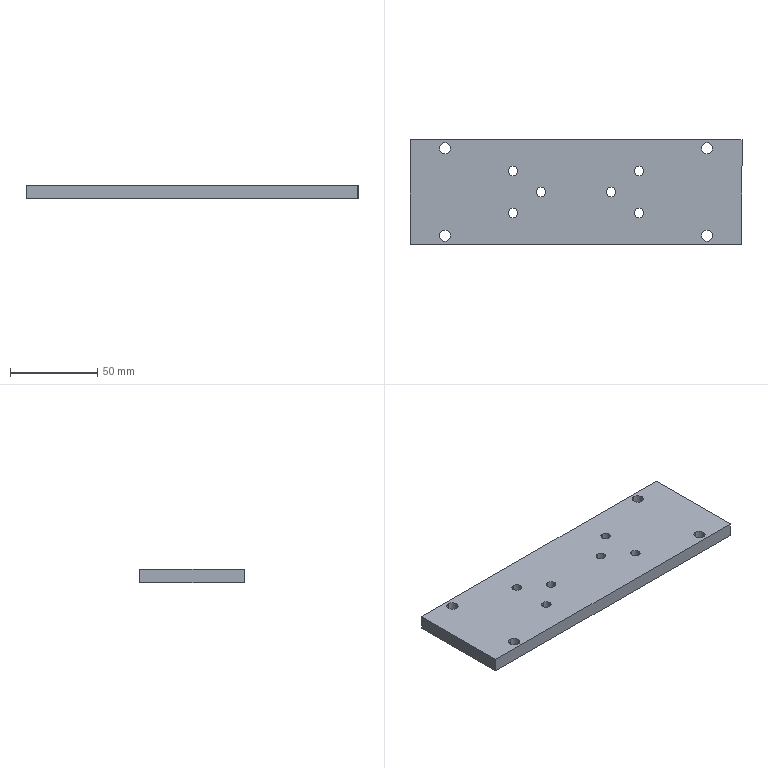Component | SolidWorks | JQ-2-0-001-1 | 1 solid | 26 faces | box 190 x 60 x 8 mm | volume 89071 mm3 | cylinder 20 | plane 6 | commonest cylinder face diameters 5.4 x12 6.4 x8
build123d program:
from build123d import *

# Parameters (mm, degrees)
SKETCH1_W           = 190
SKETCH1_H           = 8
BOSS_EXTRUDE1_DEPTH = 60
SKETCH7_R           = 3.2
CUT_EXTRUDE2_DEPTH  = 200.409
SKETCH8_R           = 2.7
CUT_EXTRUDE3_DEPTH  = 200.409


with BuildPart() as part:
    # Sketch1 → Boss-Extrude1 (new body)
    with BuildSketch(Plane.XY):
        with Locations((95, 4)):
            Rectangle(SKETCH1_W, SKETCH1_H)
    extrude(amount=BOSS_EXTRUDE1_DEPTH)

    # Sketch7 → Cut-Extrude2 (cut, through all)
    with BuildSketch(Plane(origin=(0, 8, 0), x_dir=(1, 0, 0), z_dir=(0, 1, 0))):
        with Locations(Location((170, -5, 0), (0, 0, 270))):
            Circle(SKETCH7_R)
        with Locations(Location((170, -55, 0), (0, 0, 270))):
            Circle(SKETCH7_R)
        with Locations(Location((20, -5, 0), (0, 0, 270))):
            Circle(SKETCH7_R)
        with Locations(Location((20, -55, 0), (0, 0, 270))):
            Circle(SKETCH7_R)
    extrude(amount=-CUT_EXTRUDE2_DEPTH, mode=Mode.SUBTRACT)

    # Sketch8 → Cut-Extrude3 (cut, through all)
    with BuildSketch(Plane.XZ):
        with Locations(Location((59, 42, 0), (0, 0, 270))):
            Circle(SKETCH8_R)
        with Locations(Location((131, 42, 0), (0, 0, 270))):
            Circle(SKETCH8_R)
        with Locations(Location((59, 18, 0), (0, 0, 270))):
            Circle(SKETCH8_R)
        with Locations(Location((131, 18, 0), (0, 0, 270))):
            Circle(SKETCH8_R)
        with Locations(Location((75, 30, 0), (0, 0, 270))):
            Circle(SKETCH8_R)
        with Locations(Location((115, 30, 0), (0, 0, 270))):
            Circle(SKETCH8_R)
    extrude(amount=-CUT_EXTRUDE3_DEPTH, mode=Mode.SUBTRACT)


solid = part.part

# Placed as in the assembly
solid = solid.moved(Location((-357.058, 59.339, -23.869), (90, 0, 0)))
STEP:
#1=CARTESIAN_POINT('',(-9.53,1.261,-0.9397));
#2=VERTEX_POINT('',#1);
#3=CARTESIAN_POINT('',(-9.53,1.049,-0.9397));
#4=VERTEX_POINT('',#3);
#5=CARTESIAN_POINT('',(-9.53,1.155,-0.9397));
#6=DIRECTION('',(0.,0.,1.));
#7=DIRECTION('',(0.,-1.,0.));
#8=AXIS2_PLACEMENT_3D('',#5,#6,#7);
#9=CIRCLE('',#8,0.1063);
#10=EDGE_CURVE('',#2,#4,#9,.T.);
#11=ORIENTED_EDGE('',*,*,#10,.F.);
#12=CARTESIAN_POINT('',(-9.53,1.261,-0.6248));
#13=VERTEX_POINT('',#12);
#14=CARTESIAN_POINT('',(-9.53,1.261,-0.9397));
#15=DIRECTION('',(0.,0.,1.));
#16=VECTOR('',#15,39.37);
#17=LINE('',#14,#16);
#18=EDGE_CURVE('',#2,#13,#17,.T.);
#19=ORIENTED_EDGE('',*,*,#18,.T.);
#20=CARTESIAN_POINT('',(-9.53,1.049,-0.6248));
#21=VERTEX_POINT('',#20);
#22=CARTESIAN_POINT('',(-9.53,1.155,-0.6248));
#23=DIRECTION('',(0.,0.,1.));
#24=DIRECTION('',(0.,-1.,0.));
#25=AXIS2_PLACEMENT_3D('',#22,#23,#24);
#26=CIRCLE('',#25,0.1063);
#27=EDGE_CURVE('',#13,#21,#26,.T.);
#28=ORIENTED_EDGE('',*,*,#27,.T.);
#29=CARTESIAN_POINT('',(-9.53,1.049,-0.9397));
#30=DIRECTION('',(0.,0.,1.));
#31=VECTOR('',#30,39.37);
#32=LINE('',#29,#31);
#33=EDGE_CURVE('',#4,#21,#32,.T.);
#34=ORIENTED_EDGE('',*,*,#33,.F.);
#35=EDGE_LOOP('',(#11,#19,#28,#34));
#36=FACE_OUTER_BOUND('',#35,.T.);
#37=CARTESIAN_POINT('',(-9.53,1.155,-0.9397));
#38=DIRECTION('',(0.,0.,1.));
#39=DIRECTION('',(0.,-1.,0.));
#40=AXIS2_PLACEMENT_3D('',#37,#38,#39);
#41=CYLINDRICAL_SURFACE('',#40,0.1063);
#42=ADVANCED_FACE('',(#36),#41,.F.);
#43=CARTESIAN_POINT('',(-11.105,1.261,-0.9397));
#44=VERTEX_POINT('',#43);
#45=CARTESIAN_POINT('',(-11.105,1.049,-0.9397));
#46=VERTEX_POINT('',#45);
#47=CARTESIAN_POINT('',(-11.105,1.155,-0.9397));
#48=DIRECTION('',(0.,0.,1.));
#49=DIRECTION('',(0.,-1.,0.));
#50=AXIS2_PLACEMENT_3D('',#47,#48,#49);
#51=CIRCLE('',#50,0.1063);
#52=EDGE_CURVE('',#44,#46,#51,.T.);
#53=ORIENTED_EDGE('',*,*,#52,.F.);
#54=CARTESIAN_POINT('',(-11.105,1.261,-0.6248));
#55=VERTEX_POINT('',#54);
#56=CARTESIAN_POINT('',(-11.105,1.261,-0.9397));
#57=DIRECTION('',(0.,0.,1.));
#58=VECTOR('',#57,39.37);
#59=LINE('',#56,#58);
#60=EDGE_CURVE('',#44,#55,#59,.T.);
#61=ORIENTED_EDGE('',*,*,#60,.T.);
#62=CARTESIAN_POINT('',(-11.105,1.049,-0.6248));
#63=VERTEX_POINT('',#62);
#64=CARTESIAN_POINT('',(-11.105,1.155,-0.6248));
#65=DIRECTION('',(0.,0.,1.));
#66=DIRECTION('',(0.,-1.,0.));
#67=AXIS2_PLACEMENT_3D('',#64,#65,#66);
#68=CIRCLE('',#67,0.1063);
#69=EDGE_CURVE('',#55,#63,#68,.T.);
#70=ORIENTED_EDGE('',*,*,#69,.T.);
#71=CARTESIAN_POINT('',(-11.105,1.049,-0.9397));
#72=DIRECTION('',(0.,0.,1.));
#73=VECTOR('',#72,39.37);
#74=LINE('',#71,#73);
#75=EDGE_CURVE('',#46,#63,#74,.T.);
#76=ORIENTED_EDGE('',*,*,#75,.F.);
#77=EDGE_LOOP('',(#53,#61,#70,#76));
#78=FACE_OUTER_BOUND('',#77,.T.);
#79=CARTESIAN_POINT('',(-11.105,1.155,-0.9397));
#80=DIRECTION('',(0.,0.,1.));
#81=DIRECTION('',(0.,-1.,0.));
#82=AXIS2_PLACEMENT_3D('',#79,#80,#81);
#83=CYLINDRICAL_SURFACE('',#82,0.1063);
#84=ADVANCED_FACE('',(#78),#83,.F.);
#85=CARTESIAN_POINT('',(-8.9,0.7889,-0.9397));
#86=VERTEX_POINT('',#85);
#87=CARTESIAN_POINT('',(-8.9,0.5763,-0.9397));
#88=VERTEX_POINT('',#87);
#89=CARTESIAN_POINT('',(-8.9,0.6826,-0.9397));
#90=DIRECTION('',(0.,0.,1.));
#91=DIRECTION('',(0.,-1.,0.));
#92=AXIS2_PLACEMENT_3D('',#89,#90,#91);
#93=CIRCLE('',#92,0.1063);
#94=EDGE_CURVE('',#86,#88,#93,.T.);
#95=ORIENTED_EDGE('',*,*,#94,.F.);
#96=CARTESIAN_POINT('',(-8.9,0.7889,-0.6248));
#97=VERTEX_POINT('',#96);
#98=CARTESIAN_POINT('',(-8.9,0.7889,-0.9397));
#99=DIRECTION('',(0.,0.,1.));
#100=VECTOR('',#99,39.37);
#101=LINE('',#98,#100);
#102=EDGE_CURVE('',#86,#97,#101,.T.);
#103=ORIENTED_EDGE('',*,*,#102,.T.);
#104=CARTESIAN_POINT('',(-8.9,0.5763,-0.6248));
#105=VERTEX_POINT('',#104);
#106=CARTESIAN_POINT('',(-8.9,0.6826,-0.6248));
#107=DIRECTION('',(0.,0.,1.));
#108=DIRECTION('',(0.,-1.,0.));
#109=AXIS2_PLACEMENT_3D('',#106,#107,#108);
#110=CIRCLE('',#109,0.1063);
#111=EDGE_CURVE('',#97,#105,#110,.T.);
#112=ORIENTED_EDGE('',*,*,#111,.T.);
#113=CARTESIAN_POINT('',(-8.9,0.5763,-0.9397));
#114=DIRECTION('',(0.,0.,1.));
#115=VECTOR('',#114,39.37);
#116=LINE('',#113,#115);
#117=EDGE_CURVE('',#88,#105,#116,.T.);
#118=ORIENTED_EDGE('',*,*,#117,.F.);
#119=EDGE_LOOP('',(#95,#103,#112,#118));
#120=FACE_OUTER_BOUND('',#119,.T.);
#121=CARTESIAN_POINT('',(-8.9,0.6826,-0.9397));
#122=DIRECTION('',(0.,0.,1.));
#123=DIRECTION('',(0.,-1.,0.));
#124=AXIS2_PLACEMENT_3D('',#121,#122,#123);
#125=CYLINDRICAL_SURFACE('',#124,0.1063);
#126=ADVANCED_FACE('',(#120),#125,.F.);
#127=CARTESIAN_POINT('',(-11.735,0.7889,-0.9397));
#128=VERTEX_POINT('',#127);
#129=CARTESIAN_POINT('',(-11.735,0.5763,-0.9397));
#130=VERTEX_POINT('',#129);
#131=CARTESIAN_POINT('',(-11.735,0.6826,-0.9397));
#132=DIRECTION('',(0.,0.,1.));
#133=DIRECTION('',(0.,-1.,0.));
#134=AXIS2_PLACEMENT_3D('',#131,#132,#133);
#135=CIRCLE('',#134,0.1063);
#136=EDGE_CURVE('',#128,#130,#135,.T.);
#137=ORIENTED_EDGE('',*,*,#136,.F.);
#138=CARTESIAN_POINT('',(-11.735,0.7889,-0.6248));
#139=VERTEX_POINT('',#138);
#140=CARTESIAN_POINT('',(-11.735,0.7889,-0.9397));
#141=DIRECTION('',(0.,0.,1.));
#142=VECTOR('',#141,39.37);
#143=LINE('',#140,#142);
#144=EDGE_CURVE('',#128,#139,#143,.T.);
#145=ORIENTED_EDGE('',*,*,#144,.T.);
#146=CARTESIAN_POINT('',(-11.735,0.5763,-0.6248));
#147=VERTEX_POINT('',#146);
#148=CARTESIAN_POINT('',(-11.735,0.6826,-0.6248));
#149=DIRECTION('',(0.,0.,1.));
#150=DIRECTION('',(0.,-1.,0.));
#151=AXIS2_PLACEMENT_3D('',#148,#149,#150);
#152=CIRCLE('',#151,0.1063);
#153=EDGE_CURVE('',#139,#147,#152,.T.);
#154=ORIENTED_EDGE('',*,*,#153,.T.);
#155=CARTESIAN_POINT('',(-11.735,0.5763,-0.9397));
#156=DIRECTION('',(0.,0.,1.));
#157=VECTOR('',#156,39.37);
#158=LINE('',#155,#157);
#159=EDGE_CURVE('',#130,#147,#158,.T.);
#160=ORIENTED_EDGE('',*,*,#159,.F.);
#161=EDGE_LOOP('',(#137,#145,#154,#160));
#162=FACE_OUTER_BOUND('',#161,.T.);
#163=CARTESIAN_POINT('',(-11.735,0.6826,-0.9397));
#164=DIRECTION('',(0.,0.,1.));
#165=DIRECTION('',(0.,-1.,0.));
#166=AXIS2_PLACEMENT_3D('',#163,#164,#165);
#167=CYLINDRICAL_SURFACE('',#166,0.1063);
#168=ADVANCED_FACE('',(#162),#167,.F.);
#169=CARTESIAN_POINT('',(-8.9,1.734,-0.9397));
#170=VERTEX_POINT('',#169);
#171=CARTESIAN_POINT('',(-8.9,1.521,-0.9397));
#172=VERTEX_POINT('',#171);
#173=CARTESIAN_POINT('',(-8.9,1.628,-0.9397));
#174=DIRECTION('',(0.,0.,1.));
#175=DIRECTION('',(0.,-1.,0.));
#176=AXIS2_PLACEMENT_3D('',#173,#174,#175);
#177=CIRCLE('',#176,0.1063);
#178=EDGE_CURVE('',#170,#172,#177,.T.);
#179=ORIENTED_EDGE('',*,*,#178,.F.);
#180=CARTESIAN_POINT('',(-8.9,1.734,-0.6248));
#181=VERTEX_POINT('',#180);
#182=CARTESIAN_POINT('',(-8.9,1.734,-0.9397));
#183=DIRECTION('',(0.,0.,1.));
#184=VECTOR('',#183,39.37);
#185=LINE('',#182,#184);
#186=EDGE_CURVE('',#170,#181,#185,.T.);
#187=ORIENTED_EDGE('',*,*,#186,.T.);
#188=CARTESIAN_POINT('',(-8.9,1.521,-0.6248));
#189=VERTEX_POINT('',#188);
#190=CARTESIAN_POINT('',(-8.9,1.628,-0.6248));
#191=DIRECTION('',(0.,0.,1.));
#192=DIRECTION('',(0.,-1.,0.));
#193=AXIS2_PLACEMENT_3D('',#190,#191,#192);
#194=CIRCLE('',#193,0.1063);
#195=EDGE_CURVE('',#181,#189,#194,.T.);
#196=ORIENTED_EDGE('',*,*,#195,.T.);
#197=CARTESIAN_POINT('',(-8.9,1.521,-0.9397));
#198=DIRECTION('',(0.,0.,1.));
#199=VECTOR('',#198,39.37);
#200=LINE('',#197,#199);
#201=EDGE_CURVE('',#172,#189,#200,.T.);
#202=ORIENTED_EDGE('',*,*,#201,.F.);
#203=EDGE_LOOP('',(#179,#187,#196,#202));
#204=FACE_OUTER_BOUND('',#203,.T.);
#205=CARTESIAN_POINT('',(-8.9,1.628,-0.9397));
#206=DIRECTION('',(0.,0.,1.));
#207=DIRECTION('',(0.,-1.,0.));
#208=AXIS2_PLACEMENT_3D('',#205,#206,#207);
#209=CYLINDRICAL_SURFACE('',#208,0.1063);
#210=ADVANCED_FACE('',(#204),#209,.F.);
#211=CARTESIAN_POINT('',(-11.735,1.734,-0.9397));
#212=VERTEX_POINT('',#211);
#213=CARTESIAN_POINT('',(-11.735,1.521,-0.9397));
#214=VERTEX_POINT('',#213);
#215=CARTESIAN_POINT('',(-11.735,1.628,-0.9397));
#216=DIRECTION('',(0.,0.,1.));
#217=DIRECTION('',(0.,-1.,0.));
#218=AXIS2_PLACEMENT_3D('',#215,#216,#217);
#219=CIRCLE('',#218,0.1063);
#220=EDGE_CURVE('',#212,#214,#219,.T.);
#221=ORIENTED_EDGE('',*,*,#220,.F.);
#222=CARTESIAN_POINT('',(-11.735,1.734,-0.6248));
#223=VERTEX_POINT('',#222);
#224=CARTESIAN_POINT('',(-11.735,1.734,-0.9397));
#225=DIRECTION('',(0.,0.,1.));
#226=VECTOR('',#225,39.37);
#227=LINE('',#224,#226);
#228=EDGE_CURVE('',#212,#223,#227,.T.);
#229=ORIENTED_EDGE('',*,*,#228,.T.);
#230=CARTESIAN_POINT('',(-11.735,1.521,-0.6248));
#231=VERTEX_POINT('',#230);
#232=CARTESIAN_POINT('',(-11.735,1.628,-0.6248));
#233=DIRECTION('',(0.,0.,1.));
#234=DIRECTION('',(0.,-1.,0.));
#235=AXIS2_PLACEMENT_3D('',#232,#233,#234);
#236=CIRCLE('',#235,0.1063);
#237=EDGE_CURVE('',#223,#231,#236,.T.);
#238=ORIENTED_EDGE('',*,*,#237,.T.);
#239=CARTESIAN_POINT('',(-11.735,1.521,-0.9397));
#240=DIRECTION('',(0.,0.,1.));
#241=VECTOR('',#240,39.37);
#242=LINE('',#239,#241);
#243=EDGE_CURVE('',#214,#231,#242,.T.);
#244=ORIENTED_EDGE('',*,*,#243,.F.);
#245=EDGE_LOOP('',(#221,#229,#238,#244));
#246=FACE_OUTER_BOUND('',#245,.T.);
#247=CARTESIAN_POINT('',(-11.735,1.628,-0.9397));
#248=DIRECTION('',(0.,0.,1.));
#249=DIRECTION('',(0.,-1.,0.));
#250=AXIS2_PLACEMENT_3D('',#247,#248,#249);
#251=CYLINDRICAL_SURFACE('',#250,0.1063);
#252=ADVANCED_FACE('',(#246),#251,.F.);
#253=CARTESIAN_POINT('',(-13.27,2.013,-0.6248));
#254=VERTEX_POINT('',#253);
#255=CARTESIAN_POINT('',(-13.27,2.265,-0.6248));
#256=VERTEX_POINT('',#255);
#257=CARTESIAN_POINT('',(-13.27,2.139,-0.6248));
#258=DIRECTION('',(-0.,-0.,-1.));
#259=DIRECTION('',(0.,1.,0.));
#260=AXIS2_PLACEMENT_3D('',#257,#258,#259);
#261=CIRCLE('',#260,0.126);
#262=EDGE_CURVE('',#254,#256,#261,.T.);
#263=ORIENTED_EDGE('',*,*,#262,.F.);
#264=CARTESIAN_POINT('',(-13.27,2.013,-0.9397));
#265=VERTEX_POINT('',#264);
#266=CARTESIAN_POINT('',(-13.27,2.013,-0.6248));
#267=DIRECTION('',(-0.,-0.,-1.));
#268=VECTOR('',#267,39.37);
#269=LINE('',#266,#268);
#270=EDGE_CURVE('',#254,#265,#269,.T.);
#271=ORIENTED_EDGE('',*,*,#270,.T.);
#272=CARTESIAN_POINT('',(-13.27,2.265,-0.9397));
#273=VERTEX_POINT('',#272);
#274=CARTESIAN_POINT('',(-13.27,2.139,-0.9397));
#275=DIRECTION('',(-0.,-0.,-1.));
#276=DIRECTION('',(0.,1.,0.));
#277=AXIS2_PLACEMENT_3D('',#274,#275,#276);
#278=CIRCLE('',#277,0.126);
#279=EDGE_CURVE('',#265,#273,#278,.T.);
#280=ORIENTED_EDGE('',*,*,#279,.T.);
#281=CARTESIAN_POINT('',(-13.27,2.265,-0.6248));
#282=DIRECTION('',(-0.,-0.,-1.));
#283=VECTOR('',#282,39.37);
#284=LINE('',#281,#283);
#285=EDGE_CURVE('',#256,#273,#284,.T.);
#286=ORIENTED_EDGE('',*,*,#285,.F.);
#287=EDGE_LOOP('',(#263,#271,#280,#286));
#288=FACE_OUTER_BOUND('',#287,.T.);
#289=CARTESIAN_POINT('',(-13.27,2.139,-0.6248));
#290=DIRECTION('',(-0.,-0.,-1.));
#291=DIRECTION('',(0.,1.,0.));
#292=AXIS2_PLACEMENT_3D('',#289,#290,#291);
#293=CYLINDRICAL_SURFACE('',#292,0.126);
#294=ADVANCED_FACE('',(#288),#293,.F.);
#295=CARTESIAN_POINT('',(-13.27,0.04485,-0.6248));
#296=VERTEX_POINT('',#295);
#297=CARTESIAN_POINT('',(-13.27,0.2968,-0.6248));
#298=VERTEX_POINT('',#297);
#299=CARTESIAN_POINT('',(-13.27,0.1708,-0.6248));
#300=DIRECTION('',(-0.,-0.,-1.));
#301=DIRECTION('',(0.,1.,0.));
#302=AXIS2_PLACEMENT_3D('',#299,#300,#301);
#303=CIRCLE('',#302,0.126);
#304=EDGE_CURVE('',#296,#298,#303,.T.);
#305=ORIENTED_EDGE('',*,*,#304,.F.);
#306=CARTESIAN_POINT('',(-13.27,0.04485,-0.9397));
#307=VERTEX_POINT('',#306);
#308=CARTESIAN_POINT('',(-13.27,0.04485,-0.6248));
#309=DIRECTION('',(-0.,-0.,-1.));
#310=VECTOR('',#309,39.37);
#311=LINE('',#308,#310);
#312=EDGE_CURVE('',#296,#307,#311,.T.);
#313=ORIENTED_EDGE('',*,*,#312,.T.);
#314=CARTESIAN_POINT('',(-13.27,0.2968,-0.9397));
#315=VERTEX_POINT('',#314);
#316=CARTESIAN_POINT('',(-13.27,0.1708,-0.9397));
#317=DIRECTION('',(-0.,-0.,-1.));
#318=DIRECTION('',(0.,1.,0.));
#319=AXIS2_PLACEMENT_3D('',#316,#317,#318);
#320=CIRCLE('',#319,0.126);
#321=EDGE_CURVE('',#307,#315,#320,.T.);
#322=ORIENTED_EDGE('',*,*,#321,.T.);
#323=CARTESIAN_POINT('',(-13.27,0.2968,-0.6248));
#324=DIRECTION('',(-0.,-0.,-1.));
#325=VECTOR('',#324,39.37);
#326=LINE('',#323,#325);
#327=EDGE_CURVE('',#298,#315,#326,.T.);
#328=ORIENTED_EDGE('',*,*,#327,.F.);
#329=EDGE_LOOP('',(#305,#313,#322,#328));
#330=FACE_OUTER_BOUND('',#329,.T.);
#331=CARTESIAN_POINT('',(-13.27,0.1708,-0.6248));
#332=DIRECTION('',(-0.,-0.,-1.));
#333=DIRECTION('',(0.,1.,0.));
#334=AXIS2_PLACEMENT_3D('',#331,#332,#333);
#335=CYLINDRICAL_SURFACE('',#334,0.126);
#336=ADVANCED_FACE('',(#330),#335,.F.);
#337=CARTESIAN_POINT('',(-7.365,2.013,-0.6248));
#338=VERTEX_POINT('',#337);
#339=CARTESIAN_POINT('',(-7.365,2.265,-0.6248));
#340=VERTEX_POINT('',#339);
#341=CARTESIAN_POINT('',(-7.365,2.139,-0.6248));
#342=DIRECTION('',(-0.,-0.,-1.));
#343=DIRECTION('',(0.,1.,0.));
#344=AXIS2_PLACEMENT_3D('',#341,#342,#343);
#345=CIRCLE('',#344,0.126);
#346=EDGE_CURVE('',#338,#340,#345,.T.);
#347=ORIENTED_EDGE('',*,*,#346,.F.);
#348=CARTESIAN_POINT('',(-7.365,2.013,-0.9397));
#349=VERTEX_POINT('',#348);
#350=CARTESIAN_POINT('',(-7.365,2.013,-0.6248));
#351=DIRECTION('',(-0.,-0.,-1.));
#352=VECTOR('',#351,39.37);
#353=LINE('',#350,#352);
#354=EDGE_CURVE('',#338,#349,#353,.T.);
#355=ORIENTED_EDGE('',*,*,#354,.T.);
#356=CARTESIAN_POINT('',(-7.365,2.265,-0.9397));
#357=VERTEX_POINT('',#356);
#358=CARTESIAN_POINT('',(-7.365,2.139,-0.9397));
#359=DIRECTION('',(-0.,-0.,-1.));
#360=DIRECTION('',(0.,1.,0.));
#361=AXIS2_PLACEMENT_3D('',#358,#359,#360);
#362=CIRCLE('',#361,0.126);
#363=EDGE_CURVE('',#349,#357,#362,.T.);
#364=ORIENTED_EDGE('',*,*,#363,.T.);
#365=CARTESIAN_POINT('',(-7.365,2.265,-0.6248));
#366=DIRECTION('',(-0.,-0.,-1.));
#367=VECTOR('',#366,39.37);
#368=LINE('',#365,#367);
#369=EDGE_CURVE('',#340,#357,#368,.T.);
#370=ORIENTED_EDGE('',*,*,#369,.F.);
#371=EDGE_LOOP('',(#347,#355,#364,#370));
#372=FACE_OUTER_BOUND('',#371,.T.);
#373=CARTESIAN_POINT('',(-7.365,2.139,-0.6248));
#374=DIRECTION('',(-0.,-0.,-1.));
#375=DIRECTION('',(0.,1.,0.));
#376=AXIS2_PLACEMENT_3D('',#373,#374,#375);
#377=CYLINDRICAL_SURFACE('',#376,0.126);
#378=ADVANCED_FACE('',(#372),#377,.F.);
#379=CARTESIAN_POINT('',(-7.365,0.04485,-0.6248));
#380=VERTEX_POINT('',#379);
#381=CARTESIAN_POINT('',(-7.365,0.2968,-0.6248));
#382=VERTEX_POINT('',#381);
#383=CARTESIAN_POINT('',(-7.365,0.1708,-0.6248));
#384=DIRECTION('',(-0.,-0.,-1.));
#385=DIRECTION('',(0.,1.,0.));
#386=AXIS2_PLACEMENT_3D('',#383,#384,#385);
#387=CIRCLE('',#386,0.126);
#388=EDGE_CURVE('',#380,#382,#387,.T.);
#389=ORIENTED_EDGE('',*,*,#388,.F.);
#390=CARTESIAN_POINT('',(-7.365,0.04485,-0.9397));
#391=VERTEX_POINT('',#390);
#392=CARTESIAN_POINT('',(-7.365,0.04485,-0.6248));
#393=DIRECTION('',(-0.,-0.,-1.));
#394=VECTOR('',#393,39.37);
#395=LINE('',#392,#394);
#396=EDGE_CURVE('',#380,#391,#395,.T.);
#397=ORIENTED_EDGE('',*,*,#396,.T.);
#398=CARTESIAN_POINT('',(-7.365,0.2968,-0.9397));
#399=VERTEX_POINT('',#398);
#400=CARTESIAN_POINT('',(-7.365,0.1708,-0.9397));
#401=DIRECTION('',(-0.,-0.,-1.));
#402=DIRECTION('',(0.,1.,0.));
#403=AXIS2_PLACEMENT_3D('',#400,#401,#402);
#404=CIRCLE('',#403,0.126);
#405=EDGE_CURVE('',#391,#399,#404,.T.);
#406=ORIENTED_EDGE('',*,*,#405,.T.);
#407=CARTESIAN_POINT('',(-7.365,0.2968,-0.6248));
#408=DIRECTION('',(-0.,-0.,-1.));
#409=VECTOR('',#408,39.37);
#410=LINE('',#407,#409);
#411=EDGE_CURVE('',#382,#399,#410,.T.);
#412=ORIENTED_EDGE('',*,*,#411,.F.);
#413=EDGE_LOOP('',(#389,#397,#406,#412));
#414=FACE_OUTER_BOUND('',#413,.T.);
#415=CARTESIAN_POINT('',(-7.365,0.1708,-0.6248));
#416=DIRECTION('',(-0.,-0.,-1.));
#417=DIRECTION('',(0.,1.,0.));
#418=AXIS2_PLACEMENT_3D('',#415,#416,#417);
#419=CYLINDRICAL_SURFACE('',#418,0.126);
#420=ADVANCED_FACE('',(#414),#419,.F.);
#421=CARTESIAN_POINT('',(-14.057,-0.02602,-0.9397));
#422=VERTEX_POINT('',#421);
#423=CARTESIAN_POINT('',(-14.057,-0.02602,-0.6248));
#424=VERTEX_POINT('',#423);
#425=CARTESIAN_POINT('',(-14.057,-0.02602,-0.6248));
#426=DIRECTION('',(0.,0.,1.));
#427=VECTOR('',#426,39.37);
#428=LINE('',#425,#427);
#429=EDGE_CURVE('',#422,#424,#428,.T.);
#430=ORIENTED_EDGE('',*,*,#429,.T.);
#431=CARTESIAN_POINT('',(-14.057,2.336,-0.6248));
#432=VERTEX_POINT('',#431);
#433=CARTESIAN_POINT('',(-14.057,2.336,-0.6248));
#434=DIRECTION('',(-0.,-1.,0.));
#435=VECTOR('',#434,39.37);
#436=LINE('',#433,#435);
#437=EDGE_CURVE('',#432,#424,#436,.T.);
#438=ORIENTED_EDGE('',*,*,#437,.F.);
#439=CARTESIAN_POINT('',(-14.057,2.336,-0.9397));
#440=VERTEX_POINT('',#439);
#441=CARTESIAN_POINT('',(-14.057,2.336,-0.6248));
#442=DIRECTION('',(0.,0.,1.));
#443=VECTOR('',#442,39.37);
#444=LINE('',#441,#443);
#445=EDGE_CURVE('',#440,#432,#444,.T.);
#446=ORIENTED_EDGE('',*,*,#445,.F.);
#447=CARTESIAN_POINT('',(-14.057,2.336,-0.9397));
#448=DIRECTION('',(-0.,-1.,0.));
#449=VECTOR('',#448,39.37);
#450=LINE('',#447,#449);
#451=EDGE_CURVE('',#440,#422,#450,.T.);
#452=ORIENTED_EDGE('',*,*,#451,.T.);
#453=EDGE_LOOP('',(#430,#438,#446,#452));
#454=FACE_OUTER_BOUND('',#453,.T.);
#455=CARTESIAN_POINT('',(-14.057,2.336,-0.6248));
#456=DIRECTION('',(1.,-0.,-0.));
#457=DIRECTION('',(-0.,-1.,0.));
#458=AXIS2_PLACEMENT_3D('',#455,#456,#457);
#459=PLANE('',#458);
#460=ADVANCED_FACE('',(#454),#459,.F.);
#461=CARTESIAN_POINT('',(-9.53,1.155,-0.6248));
#462=DIRECTION('',(0.,0.,1.));
#463=DIRECTION('',(0.,-1.,0.));
#464=AXIS2_PLACEMENT_3D('',#461,#462,#463);
#465=CIRCLE('',#464,0.1063);
#466=EDGE_CURVE('',#21,#13,#465,.T.);
#467=ORIENTED_EDGE('',*,*,#466,.F.);
#468=ORIENTED_EDGE('',*,*,#27,.F.);
#469=EDGE_LOOP('',(#467,#468));
#470=FACE_BOUND('',#469,.T.);
#471=CARTESIAN_POINT('',(-11.105,1.155,-0.6248));
#472=DIRECTION('',(0.,0.,1.));
#473=DIRECTION('',(0.,-1.,0.));
#474=AXIS2_PLACEMENT_3D('',#471,#472,#473);
#475=CIRCLE('',#474,0.1063);
#476=EDGE_CURVE('',#63,#55,#475,.T.);
#477=ORIENTED_EDGE('',*,*,#476,.F.);
#478=ORIENTED_EDGE('',*,*,#69,.F.);
#479=EDGE_LOOP('',(#477,#478));
#480=FACE_BOUND('',#479,.T.);
#481=CARTESIAN_POINT('',(-8.9,0.6826,-0.6248));
#482=DIRECTION('',(0.,0.,1.));
#483=DIRECTION('',(0.,-1.,0.));
#484=AXIS2_PLACEMENT_3D('',#481,#482,#483);
#485=CIRCLE('',#484,0.1063);
#486=EDGE_CURVE('',#105,#97,#485,.T.);
#487=ORIENTED_EDGE('',*,*,#486,.F.);
#488=ORIENTED_EDGE('',*,*,#111,.F.);
#489=EDGE_LOOP('',(#487,#488));
#490=FACE_BOUND('',#489,.T.);
#491=CARTESIAN_POINT('',(-11.735,0.6826,-0.6248));
#492=DIRECTION('',(0.,0.,1.));
#493=DIRECTION('',(0.,-1.,0.));
#494=AXIS2_PLACEMENT_3D('',#491,#492,#493);
#495=CIRCLE('',#494,0.1063);
#496=EDGE_CURVE('',#147,#139,#495,.T.);
#497=ORIENTED_EDGE('',*,*,#496,.F.);
#498=ORIENTED_EDGE('',*,*,#153,.F.);
#499=EDGE_LOOP('',(#497,#498));
#500=FACE_BOUND('',#499,.T.);
#501=CARTESIAN_POINT('',(-8.9,1.628,-0.6248));
#502=DIRECTION('',(0.,0.,1.));
#503=DIRECTION('',(0.,-1.,0.));
#504=AXIS2_PLACEMENT_3D('',#501,#502,#503);
#505=CIRCLE('',#504,0.1063);
#506=EDGE_CURVE('',#189,#181,#505,.T.);
#507=ORIENTED_EDGE('',*,*,#506,.F.);
#508=ORIENTED_EDGE('',*,*,#195,.F.);
#509=EDGE_LOOP('',(#507,#508));
#510=FACE_BOUND('',#509,.T.);
#511=CARTESIAN_POINT('',(-11.735,1.628,-0.6248));
#512=DIRECTION('',(0.,0.,1.));
#513=DIRECTION('',(0.,-1.,0.));
#514=AXIS2_PLACEMENT_3D('',#511,#512,#513);
#515=CIRCLE('',#514,0.1063);
#516=EDGE_CURVE('',#231,#223,#515,.T.);
#517=ORIENTED_EDGE('',*,*,#516,.F.);
#518=ORIENTED_EDGE('',*,*,#237,.F.);
#519=EDGE_LOOP('',(#517,#518));
#520=FACE_BOUND('',#519,.T.);
#521=CARTESIAN_POINT('',(-13.27,2.139,-0.6248));
#522=DIRECTION('',(-0.,-0.,-1.));
#523=DIRECTION('',(0.,1.,0.));
#524=AXIS2_PLACEMENT_3D('',#521,#522,#523);
#525=CIRCLE('',#524,0.126);
#526=EDGE_CURVE('',#256,#254,#525,.T.);
#527=ORIENTED_EDGE('',*,*,#526,.T.);
#528=ORIENTED_EDGE('',*,*,#262,.T.);
#529=EDGE_LOOP('',(#527,#528));
#530=FACE_BOUND('',#529,.T.);
#531=CARTESIAN_POINT('',(-13.27,0.1708,-0.6248));
#532=DIRECTION('',(-0.,-0.,-1.));
#533=DIRECTION('',(0.,1.,0.));
#534=AXIS2_PLACEMENT_3D('',#531,#532,#533);
#535=CIRCLE('',#534,0.126);
#536=EDGE_CURVE('',#298,#296,#535,.T.);
#537=ORIENTED_EDGE('',*,*,#536,.T.);
#538=ORIENTED_EDGE('',*,*,#304,.T.);
#539=EDGE_LOOP('',(#537,#538));
#540=FACE_BOUND('',#539,.T.);
#541=CARTESIAN_POINT('',(-7.365,2.139,-0.6248));
#542=DIRECTION('',(-0.,-0.,-1.));
#543=DIRECTION('',(0.,1.,0.));
#544=AXIS2_PLACEMENT_3D('',#541,#542,#543);
#545=CIRCLE('',#544,0.126);
#546=EDGE_CURVE('',#340,#338,#545,.T.);
#547=ORIENTED_EDGE('',*,*,#546,.T.);
#548=ORIENTED_EDGE('',*,*,#346,.T.);
#549=EDGE_LOOP('',(#547,#548));
#550=FACE_BOUND('',#549,.T.);
#551=CARTESIAN_POINT('',(-7.365,0.1708,-0.6248));
#552=DIRECTION('',(-0.,-0.,-1.));
#553=DIRECTION('',(0.,1.,0.));
#554=AXIS2_PLACEMENT_3D('',#551,#552,#553);
#555=CIRCLE('',#554,0.126);
#556=EDGE_CURVE('',#382,#380,#555,.T.);
#557=ORIENTED_EDGE('',*,*,#556,.T.);
#558=ORIENTED_EDGE('',*,*,#388,.T.);
#559=EDGE_LOOP('',(#557,#558));
#560=FACE_BOUND('',#559,.T.);
#561=CARTESIAN_POINT('',(-6.577,-0.02602,-0.6248));
#562=VERTEX_POINT('',#561);
#563=CARTESIAN_POINT('',(-14.057,-0.02602,-0.6248));
#564=DIRECTION('',(1.,-0.,-0.));
#565=VECTOR('',#564,39.37);
#566=LINE('',#563,#565);
#567=EDGE_CURVE('',#424,#562,#566,.T.);
#568=ORIENTED_EDGE('',*,*,#567,.T.);
#569=CARTESIAN_POINT('',(-6.577,2.336,-0.6248));
#570=VERTEX_POINT('',#569);
#571=CARTESIAN_POINT('',(-6.577,2.336,-0.6248));
#572=DIRECTION('',(-0.,-1.,0.));
#573=VECTOR('',#572,39.37);
#574=LINE('',#571,#573);
#575=EDGE_CURVE('',#570,#562,#574,.T.);
#576=ORIENTED_EDGE('',*,*,#575,.F.);
#577=CARTESIAN_POINT('',(-14.057,2.336,-0.6248));
#578=DIRECTION('',(1.,-0.,-0.));
#579=VECTOR('',#578,39.37);
#580=LINE('',#577,#579);
#581=EDGE_CURVE('',#432,#570,#580,.T.);
#582=ORIENTED_EDGE('',*,*,#581,.F.);
#583=ORIENTED_EDGE('',*,*,#437,.T.);
#584=EDGE_LOOP('',(#568,#576,#582,#583));
#585=FACE_OUTER_BOUND('',#584,.T.);
#586=CARTESIAN_POINT('',(-14.057,2.336,-0.6248));
#587=DIRECTION('',(-0.,-0.,-1.));
#588=DIRECTION('',(0.,1.,-0.));
#589=AXIS2_PLACEMENT_3D('',#586,#587,#588);
#590=PLANE('',#589);
#591=ADVANCED_FACE('',(#470,#480,#490,#500,#510,#520,#530,#540,#550,#560,#585),#590,.F.);
#592=CARTESIAN_POINT('',(-6.577,-0.02602,-0.9397));
#593=VERTEX_POINT('',#592);
#594=CARTESIAN_POINT('',(-6.577,-0.02602,-0.6248));
#595=DIRECTION('',(-0.,-0.,-1.));
#596=VECTOR('',#595,39.37);
#597=LINE('',#594,#596);
#598=EDGE_CURVE('',#562,#593,#597,.T.);
#599=ORIENTED_EDGE('',*,*,#598,.T.);
#600=CARTESIAN_POINT('',(-6.577,2.336,-0.9397));
#601=VERTEX_POINT('',#600);
#602=CARTESIAN_POINT('',(-6.577,2.336,-0.9397));
#603=DIRECTION('',(-0.,-1.,0.));
#604=VECTOR('',#603,39.37);
#605=LINE('',#602,#604);
#606=EDGE_CURVE('',#601,#593,#605,.T.);
#607=ORIENTED_EDGE('',*,*,#606,.F.);
#608=CARTESIAN_POINT('',(-6.577,2.336,-0.6248));
#609=DIRECTION('',(-0.,-0.,-1.));
#610=VECTOR('',#609,39.37);
#611=LINE('',#608,#610);
#612=EDGE_CURVE('',#570,#601,#611,.T.);
#613=ORIENTED_EDGE('',*,*,#612,.F.);
#614=ORIENTED_EDGE('',*,*,#575,.T.);
#615=EDGE_LOOP('',(#599,#607,#613,#614));
#616=FACE_OUTER_BOUND('',#615,.T.);
#617=CARTESIAN_POINT('',(-6.577,2.336,-0.6248));
#618=DIRECTION('',(-1.,0.,0.));
#619=DIRECTION('',(0.,1.,-0.));
#620=AXIS2_PLACEMENT_3D('',#617,#618,#619);
#621=PLANE('',#620);
#622=ADVANCED_FACE('',(#616),#621,.F.);
#623=CARTESIAN_POINT('',(-9.53,1.155,-0.9397));
#624=DIRECTION('',(0.,0.,1.));
#625=DIRECTION('',(0.,-1.,0.));
#626=AXIS2_PLACEMENT_3D('',#623,#624,#625);
#627=CIRCLE('',#626,0.1063);
#628=EDGE_CURVE('',#4,#2,#627,.T.);
#629=ORIENTED_EDGE('',*,*,#628,.T.);
#630=ORIENTED_EDGE('',*,*,#10,.T.);
#631=EDGE_LOOP('',(#629,#630));
#632=FACE_BOUND('',#631,.T.);
#633=CARTESIAN_POINT('',(-11.105,1.155,-0.9397));
#634=DIRECTION('',(0.,0.,1.));
#635=DIRECTION('',(0.,-1.,0.));
#636=AXIS2_PLACEMENT_3D('',#633,#634,#635);
#637=CIRCLE('',#636,0.1063);
#638=EDGE_CURVE('',#46,#44,#637,.T.);
#639=ORIENTED_EDGE('',*,*,#638,.T.);
#640=ORIENTED_EDGE('',*,*,#52,.T.);
#641=EDGE_LOOP('',(#639,#640));
#642=FACE_BOUND('',#641,.T.);
#643=CARTESIAN_POINT('',(-8.9,0.6826,-0.9397));
#644=DIRECTION('',(0.,0.,1.));
#645=DIRECTION('',(0.,-1.,0.));
#646=AXIS2_PLACEMENT_3D('',#643,#644,#645);
#647=CIRCLE('',#646,0.1063);
#648=EDGE_CURVE('',#88,#86,#647,.T.);
#649=ORIENTED_EDGE('',*,*,#648,.T.);
#650=ORIENTED_EDGE('',*,*,#94,.T.);
#651=EDGE_LOOP('',(#649,#650));
#652=FACE_BOUND('',#651,.T.);
#653=CARTESIAN_POINT('',(-11.735,0.6826,-0.9397));
#654=DIRECTION('',(0.,0.,1.));
#655=DIRECTION('',(0.,-1.,0.));
#656=AXIS2_PLACEMENT_3D('',#653,#654,#655);
#657=CIRCLE('',#656,0.1063);
#658=EDGE_CURVE('',#130,#128,#657,.T.);
#659=ORIENTED_EDGE('',*,*,#658,.T.);
#660=ORIENTED_EDGE('',*,*,#136,.T.);
#661=EDGE_LOOP('',(#659,#660));
#662=FACE_BOUND('',#661,.T.);
#663=CARTESIAN_POINT('',(-8.9,1.628,-0.9397));
#664=DIRECTION('',(0.,0.,1.));
#665=DIRECTION('',(0.,-1.,0.));
#666=AXIS2_PLACEMENT_3D('',#663,#664,#665);
#667=CIRCLE('',#666,0.1063);
#668=EDGE_CURVE('',#172,#170,#667,.T.);
#669=ORIENTED_EDGE('',*,*,#668,.T.);
#670=ORIENTED_EDGE('',*,*,#178,.T.);
#671=EDGE_LOOP('',(#669,#670));
#672=FACE_BOUND('',#671,.T.);
#673=CARTESIAN_POINT('',(-11.735,1.628,-0.9397));
#674=DIRECTION('',(0.,0.,1.));
#675=DIRECTION('',(0.,-1.,0.));
#676=AXIS2_PLACEMENT_3D('',#673,#674,#675);
#677=CIRCLE('',#676,0.1063);
#678=EDGE_CURVE('',#214,#212,#677,.T.);
#679=ORIENTED_EDGE('',*,*,#678,.T.);
#680=ORIENTED_EDGE('',*,*,#220,.T.);
#681=EDGE_LOOP('',(#679,#680));
#682=FACE_BOUND('',#681,.T.);
#683=CARTESIAN_POINT('',(-13.27,2.139,-0.9397));
#684=DIRECTION('',(-0.,-0.,-1.));
#685=DIRECTION('',(0.,1.,0.));
#686=AXIS2_PLACEMENT_3D('',#683,#684,#685);
#687=CIRCLE('',#686,0.126);
#688=EDGE_CURVE('',#273,#265,#687,.T.);
#689=ORIENTED_EDGE('',*,*,#688,.F.);
#690=ORIENTED_EDGE('',*,*,#279,.F.);
#691=EDGE_LOOP('',(#689,#690));
#692=FACE_BOUND('',#691,.T.);
#693=CARTESIAN_POINT('',(-13.27,0.1708,-0.9397));
#694=DIRECTION('',(-0.,-0.,-1.));
#695=DIRECTION('',(0.,1.,0.));
#696=AXIS2_PLACEMENT_3D('',#693,#694,#695);
#697=CIRCLE('',#696,0.126);
#698=EDGE_CURVE('',#315,#307,#697,.T.);
#699=ORIENTED_EDGE('',*,*,#698,.F.);
#700=ORIENTED_EDGE('',*,*,#321,.F.);
#701=EDGE_LOOP('',(#699,#700));
#702=FACE_BOUND('',#701,.T.);
#703=CARTESIAN_POINT('',(-7.365,2.139,-0.9397));
#704=DIRECTION('',(-0.,-0.,-1.));
#705=DIRECTION('',(0.,1.,0.));
#706=AXIS2_PLACEMENT_3D('',#703,#704,#705);
#707=CIRCLE('',#706,0.126);
#708=EDGE_CURVE('',#357,#349,#707,.T.);
#709=ORIENTED_EDGE('',*,*,#708,.F.);
#710=ORIENTED_EDGE('',*,*,#363,.F.);
#711=EDGE_LOOP('',(#709,#710));
#712=FACE_BOUND('',#711,.T.);
#713=CARTESIAN_POINT('',(-7.365,0.1708,-0.9397));
#714=DIRECTION('',(-0.,-0.,-1.));
#715=DIRECTION('',(0.,1.,0.));
#716=AXIS2_PLACEMENT_3D('',#713,#714,#715);
#717=CIRCLE('',#716,0.126);
#718=EDGE_CURVE('',#399,#391,#717,.T.);
#719=ORIENTED_EDGE('',*,*,#718,.F.);
#720=ORIENTED_EDGE('',*,*,#405,.F.);
#721=EDGE_LOOP('',(#719,#720));
#722=FACE_BOUND('',#721,.T.);
#723=CARTESIAN_POINT('',(-14.057,-0.02602,-0.9397));
#724=DIRECTION('',(-1.,0.,0.));
#725=VECTOR('',#724,39.37);
#726=LINE('',#723,#725);
#727=EDGE_CURVE('',#593,#422,#726,.T.);
#728=ORIENTED_EDGE('',*,*,#727,.T.);
#729=ORIENTED_EDGE('',*,*,#451,.F.);
#730=CARTESIAN_POINT('',(-14.057,2.336,-0.9397));
#731=DIRECTION('',(-1.,0.,0.));
#732=VECTOR('',#731,39.37);
#733=LINE('',#730,#732);
#734=EDGE_CURVE('',#601,#440,#733,.T.);
#735=ORIENTED_EDGE('',*,*,#734,.F.);
#736=ORIENTED_EDGE('',*,*,#606,.T.);
#737=EDGE_LOOP('',(#728,#729,#735,#736));
#738=FACE_OUTER_BOUND('',#737,.T.);
#739=CARTESIAN_POINT('',(-14.057,2.336,-0.9397));
#740=DIRECTION('',(0.,0.,1.));
#741=DIRECTION('',(-0.,-1.,0.));
#742=AXIS2_PLACEMENT_3D('',#739,#740,#741);
#743=PLANE('',#742);
#744=ADVANCED_FACE('',(#632,#642,#652,#662,#672,#682,#692,#702,#712,#722,#738),#743,.F.);
#745=ORIENTED_EDGE('',*,*,#445,.T.);
#746=ORIENTED_EDGE('',*,*,#581,.T.);
#747=ORIENTED_EDGE('',*,*,#612,.T.);
#748=ORIENTED_EDGE('',*,*,#734,.T.);
#749=EDGE_LOOP('',(#745,#746,#747,#748));
#750=FACE_OUTER_BOUND('',#749,.T.);
#751=CARTESIAN_POINT('',(-14.057,2.336,-0.9397));
#752=DIRECTION('',(-0.,-1.,0.));
#753=DIRECTION('',(-1.,0.,0.));
#754=AXIS2_PLACEMENT_3D('',#751,#752,#753);
#755=PLANE('',#754);
#756=ADVANCED_FACE('',(#750),#755,.F.);
#757=ORIENTED_EDGE('',*,*,#429,.F.);
#758=ORIENTED_EDGE('',*,*,#727,.F.);
#759=ORIENTED_EDGE('',*,*,#598,.F.);
#760=ORIENTED_EDGE('',*,*,#567,.F.);
#761=EDGE_LOOP('',(#757,#758,#759,#760));
#762=FACE_OUTER_BOUND('',#761,.T.);
#763=CARTESIAN_POINT('',(-14.057,-0.02602,-0.9397));
#764=DIRECTION('',(-0.,-1.,0.));
#765=DIRECTION('',(-1.,0.,0.));
#766=AXIS2_PLACEMENT_3D('',#763,#764,#765);
#767=PLANE('',#766);
#768=ADVANCED_FACE('',(#762),#767,.T.);
#769=ORIENTED_EDGE('',*,*,#396,.F.);
#770=ORIENTED_EDGE('',*,*,#556,.F.);
#771=ORIENTED_EDGE('',*,*,#411,.T.);
#772=ORIENTED_EDGE('',*,*,#718,.T.);
#773=EDGE_LOOP('',(#769,#770,#771,#772));
#774=FACE_OUTER_BOUND('',#773,.T.);
#775=CARTESIAN_POINT('',(-7.365,0.1708,-0.6248));
#776=DIRECTION('',(-0.,-0.,-1.));
#777=DIRECTION('',(0.,1.,0.));
#778=AXIS2_PLACEMENT_3D('',#775,#776,#777);
#779=CYLINDRICAL_SURFACE('',#778,0.126);
#780=ADVANCED_FACE('',(#774),#779,.F.);
#781=ORIENTED_EDGE('',*,*,#354,.F.);
#782=ORIENTED_EDGE('',*,*,#546,.F.);
#783=ORIENTED_EDGE('',*,*,#369,.T.);
#784=ORIENTED_EDGE('',*,*,#708,.T.);
#785=EDGE_LOOP('',(#781,#782,#783,#784));
#786=FACE_OUTER_BOUND('',#785,.T.);
#787=CARTESIAN_POINT('',(-7.365,2.139,-0.6248));
#788=DIRECTION('',(-0.,-0.,-1.));
#789=DIRECTION('',(0.,1.,0.));
#790=AXIS2_PLACEMENT_3D('',#787,#788,#789);
#791=CYLINDRICAL_SURFACE('',#790,0.126);
#792=ADVANCED_FACE('',(#786),#791,.F.);
#793=ORIENTED_EDGE('',*,*,#312,.F.);
#794=ORIENTED_EDGE('',*,*,#536,.F.);
#795=ORIENTED_EDGE('',*,*,#327,.T.);
#796=ORIENTED_EDGE('',*,*,#698,.T.);
#797=EDGE_LOOP('',(#793,#794,#795,#796));
#798=FACE_OUTER_BOUND('',#797,.T.);
#799=CARTESIAN_POINT('',(-13.27,0.1708,-0.6248));
#800=DIRECTION('',(-0.,-0.,-1.));
#801=DIRECTION('',(0.,1.,0.));
#802=AXIS2_PLACEMENT_3D('',#799,#800,#801);
#803=CYLINDRICAL_SURFACE('',#802,0.126);
#804=ADVANCED_FACE('',(#798),#803,.F.);
#805=ORIENTED_EDGE('',*,*,#270,.F.);
#806=ORIENTED_EDGE('',*,*,#526,.F.);
#807=ORIENTED_EDGE('',*,*,#285,.T.);
#808=ORIENTED_EDGE('',*,*,#688,.T.);
#809=EDGE_LOOP('',(#805,#806,#807,#808));
#810=FACE_OUTER_BOUND('',#809,.T.);
#811=CARTESIAN_POINT('',(-13.27,2.139,-0.6248));
#812=DIRECTION('',(-0.,-0.,-1.));
#813=DIRECTION('',(0.,1.,0.));
#814=AXIS2_PLACEMENT_3D('',#811,#812,#813);
#815=CYLINDRICAL_SURFACE('',#814,0.126);
#816=ADVANCED_FACE('',(#810),#815,.F.);
#817=ORIENTED_EDGE('',*,*,#228,.F.);
#818=ORIENTED_EDGE('',*,*,#678,.F.);
#819=ORIENTED_EDGE('',*,*,#243,.T.);
#820=ORIENTED_EDGE('',*,*,#516,.T.);
#821=EDGE_LOOP('',(#817,#818,#819,#820));
#822=FACE_OUTER_BOUND('',#821,.T.);
#823=CARTESIAN_POINT('',(-11.735,1.628,-0.9397));
#824=DIRECTION('',(0.,0.,1.));
#825=DIRECTION('',(0.,-1.,0.));
#826=AXIS2_PLACEMENT_3D('',#823,#824,#825);
#827=CYLINDRICAL_SURFACE('',#826,0.1063);
#828=ADVANCED_FACE('',(#822),#827,.F.);
#829=ORIENTED_EDGE('',*,*,#186,.F.);
#830=ORIENTED_EDGE('',*,*,#668,.F.);
#831=ORIENTED_EDGE('',*,*,#201,.T.);
#832=ORIENTED_EDGE('',*,*,#506,.T.);
#833=EDGE_LOOP('',(#829,#830,#831,#832));
#834=FACE_OUTER_BOUND('',#833,.T.);
#835=CARTESIAN_POINT('',(-8.9,1.628,-0.9397));
#836=DIRECTION('',(0.,0.,1.));
#837=DIRECTION('',(0.,-1.,0.));
#838=AXIS2_PLACEMENT_3D('',#835,#836,#837);
#839=CYLINDRICAL_SURFACE('',#838,0.1063);
#840=ADVANCED_FACE('',(#834),#839,.F.);
#841=ORIENTED_EDGE('',*,*,#144,.F.);
#842=ORIENTED_EDGE('',*,*,#658,.F.);
#843=ORIENTED_EDGE('',*,*,#159,.T.);
#844=ORIENTED_EDGE('',*,*,#496,.T.);
#845=EDGE_LOOP('',(#841,#842,#843,#844));
#846=FACE_OUTER_BOUND('',#845,.T.);
#847=CARTESIAN_POINT('',(-11.735,0.6826,-0.9397));
#848=DIRECTION('',(0.,0.,1.));
#849=DIRECTION('',(0.,-1.,0.));
#850=AXIS2_PLACEMENT_3D('',#847,#848,#849);
#851=CYLINDRICAL_SURFACE('',#850,0.1063);
#852=ADVANCED_FACE('',(#846),#851,.F.);
#853=ORIENTED_EDGE('',*,*,#102,.F.);
#854=ORIENTED_EDGE('',*,*,#648,.F.);
#855=ORIENTED_EDGE('',*,*,#117,.T.);
#856=ORIENTED_EDGE('',*,*,#486,.T.);
#857=EDGE_LOOP('',(#853,#854,#855,#856));
#858=FACE_OUTER_BOUND('',#857,.T.);
#859=CARTESIAN_POINT('',(-8.9,0.6826,-0.9397));
#860=DIRECTION('',(0.,0.,1.));
#861=DIRECTION('',(0.,-1.,0.));
#862=AXIS2_PLACEMENT_3D('',#859,#860,#861);
#863=CYLINDRICAL_SURFACE('',#862,0.1063);
#864=ADVANCED_FACE('',(#858),#863,.F.);
#865=ORIENTED_EDGE('',*,*,#60,.F.);
#866=ORIENTED_EDGE('',*,*,#638,.F.);
#867=ORIENTED_EDGE('',*,*,#75,.T.);
#868=ORIENTED_EDGE('',*,*,#476,.T.);
#869=EDGE_LOOP('',(#865,#866,#867,#868));
#870=FACE_OUTER_BOUND('',#869,.T.);
#871=CARTESIAN_POINT('',(-11.105,1.155,-0.9397));
#872=DIRECTION('',(0.,0.,1.));
#873=DIRECTION('',(0.,-1.,0.));
#874=AXIS2_PLACEMENT_3D('',#871,#872,#873);
#875=CYLINDRICAL_SURFACE('',#874,0.1063);
#876=ADVANCED_FACE('',(#870),#875,.F.);
#877=ORIENTED_EDGE('',*,*,#18,.F.);
#878=ORIENTED_EDGE('',*,*,#628,.F.);
#879=ORIENTED_EDGE('',*,*,#33,.T.);
#880=ORIENTED_EDGE('',*,*,#466,.T.);
#881=EDGE_LOOP('',(#877,#878,#879,#880));
#882=FACE_OUTER_BOUND('',#881,.T.);
#883=CARTESIAN_POINT('',(-9.53,1.155,-0.9397));
#884=DIRECTION('',(0.,0.,1.));
#885=DIRECTION('',(0.,-1.,0.));
#886=AXIS2_PLACEMENT_3D('',#883,#884,#885);
#887=CYLINDRICAL_SURFACE('',#886,0.1063);
#888=ADVANCED_FACE('',(#882),#887,.F.);
#889=CLOSED_SHELL('',(#42,#84,#126,#168,#210,#252,#294,#336,#378,#420,#460,#591,#622,#744,#756,#768,#780,#792,#804,#816,#828,#840,#852,#864,#876,#888));
#890=MANIFOLD_SOLID_BREP('',#889);
#891=CARTESIAN_POINT('',(0.,0.,0.));
#892=DIRECTION('',(0.,0.,1.));
#893=DIRECTION('',(1.,0.,0.));
#894=AXIS2_PLACEMENT_3D('',#891,#892,#893);
#895=(LENGTH_UNIT()NAMED_UNIT(*)SI_UNIT($,.METRE.));
#896=LENGTH_MEASURE_WITH_UNIT(LENGTH_MEASURE(0.0254),#895);
#897=DIMENSIONAL_EXPONENTS(1.,0.,0.,0.,0.,0.,0.);
#898=(CONVERSION_BASED_UNIT('',#896)LENGTH_UNIT()NAMED_UNIT(#897));
#899=UNCERTAINTY_MEASURE_WITH_UNIT(LENGTH_MEASURE(0.00001),#898,'','');
#900=(NAMED_UNIT(*)PLANE_ANGLE_UNIT()SI_UNIT($,.RADIAN.));
#901=(NAMED_UNIT(*)SI_UNIT($,.STERADIAN.)SOLID_ANGLE_UNIT());
#902=(GEOMETRIC_REPRESENTATION_CONTEXT(3)GLOBAL_UNCERTAINTY_ASSIGNED_CONTEXT((#899))GLOBAL_UNIT_ASSIGNED_CONTEXT((#898,#900,#901))REPRESENTATION_CONTEXT('',''));
#903=ADVANCED_BREP_SHAPE_REPRESENTATION('',(#890,#894),#902);
#904=COLOUR_RGB('',0.7922,0.8196,0.9333);
#905=FILL_AREA_STYLE_COLOUR('',#904);
#906=FILL_AREA_STYLE('',(#905));
#907=SURFACE_STYLE_FILL_AREA(#906);
#908=SURFACE_SIDE_STYLE('',(#907));
#909=SURFACE_STYLE_USAGE(.BOTH.,#908);
#910=PRESENTATION_STYLE_ASSIGNMENT((#909));
#911=STYLED_ITEM('',(#910),#890);
#912=PRESENTATION_LAYER_ASSIGNMENT('','',(#911));
#913=(LENGTH_UNIT()NAMED_UNIT(*)SI_UNIT($,.METRE.));
#914=LENGTH_MEASURE_WITH_UNIT(LENGTH_MEASURE(0.0254),#913);
#915=DIMENSIONAL_EXPONENTS(1.,0.,0.,0.,0.,0.,0.);
#916=(CONVERSION_BASED_UNIT('',#914)LENGTH_UNIT()NAMED_UNIT(#915));
#917=UNCERTAINTY_MEASURE_WITH_UNIT(LENGTH_MEASURE(0.00001),#916,'','');
#918=(NAMED_UNIT(*)PLANE_ANGLE_UNIT()SI_UNIT($,.RADIAN.));
#919=(NAMED_UNIT(*)SI_UNIT($,.STERADIAN.)SOLID_ANGLE_UNIT());
#920=(GEOMETRIC_REPRESENTATION_CONTEXT(3)GLOBAL_UNCERTAINTY_ASSIGNED_CONTEXT((#917))GLOBAL_UNIT_ASSIGNED_CONTEXT((#916,#918,#919))REPRESENTATION_CONTEXT('',''));
#921=MECHANICAL_DESIGN_GEOMETRIC_PRESENTATION_REPRESENTATION('',(#911),#920);